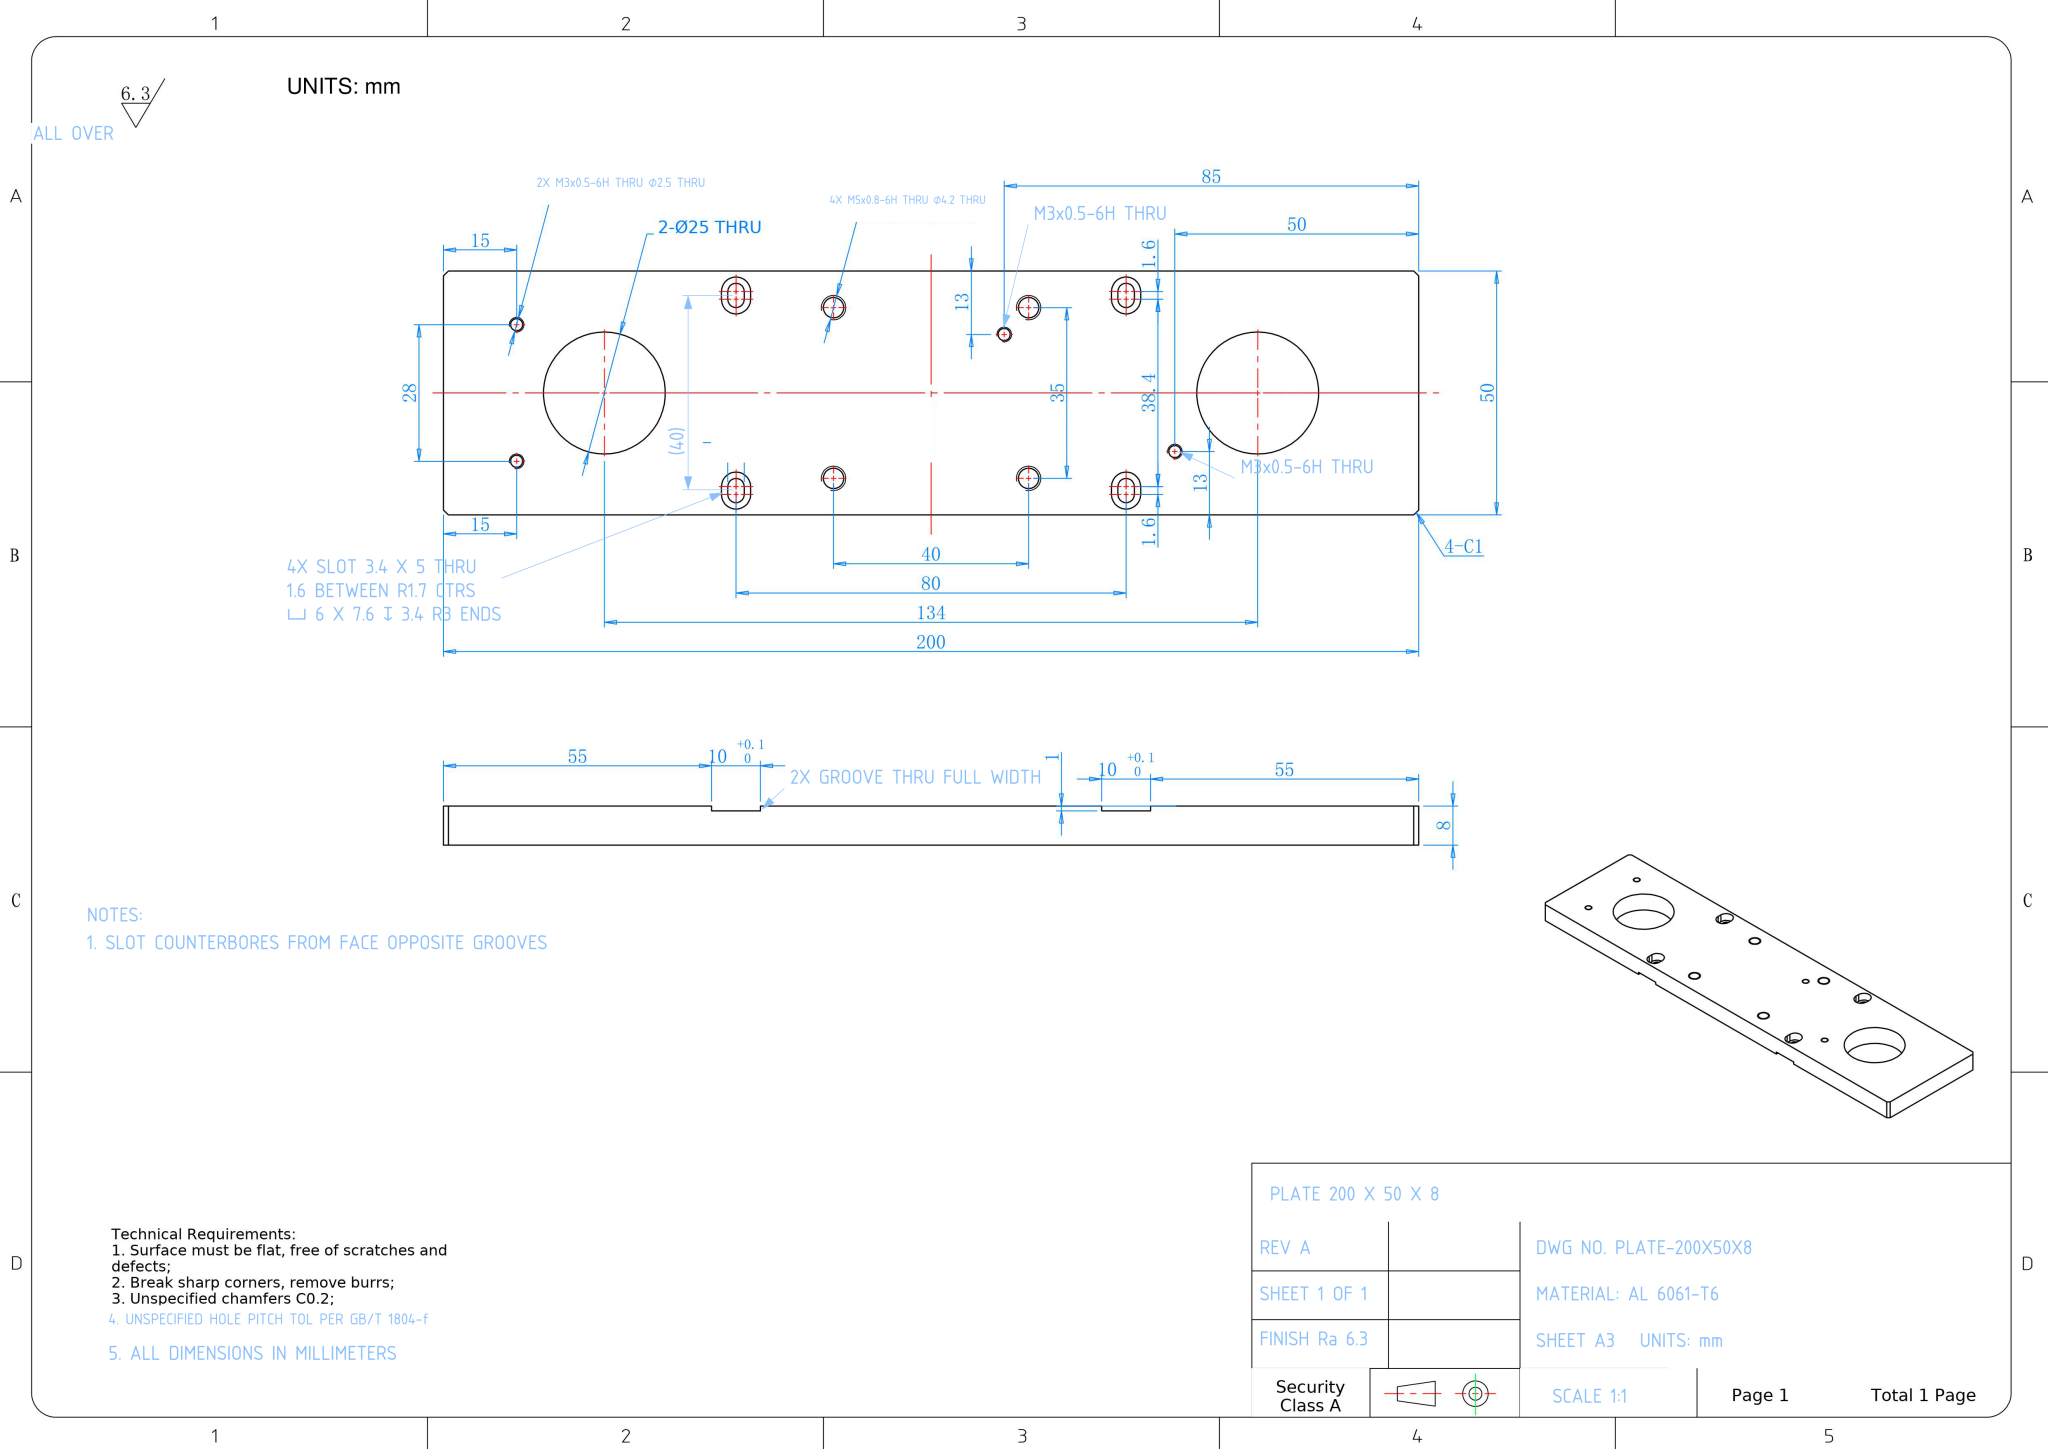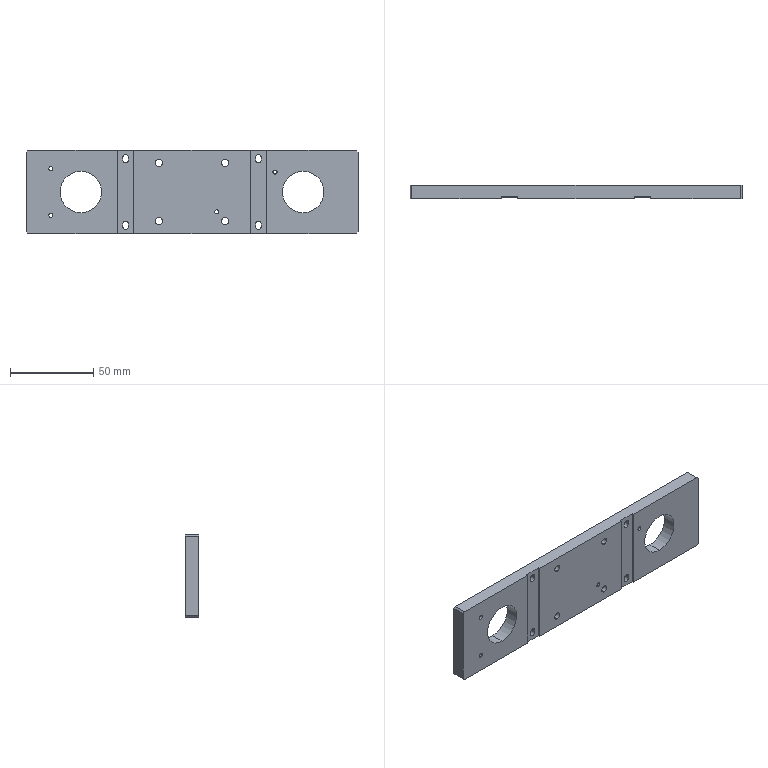Part | NX | mm | 1 solid | 82 faces | box 200 x 8 x 50 mm | volume 69805 mm3 | cylinder 44 | plane 38 | commonest cylinder face diameters 6 x12 3.4 x12 4.2 x8 2.5 x8 25 x4